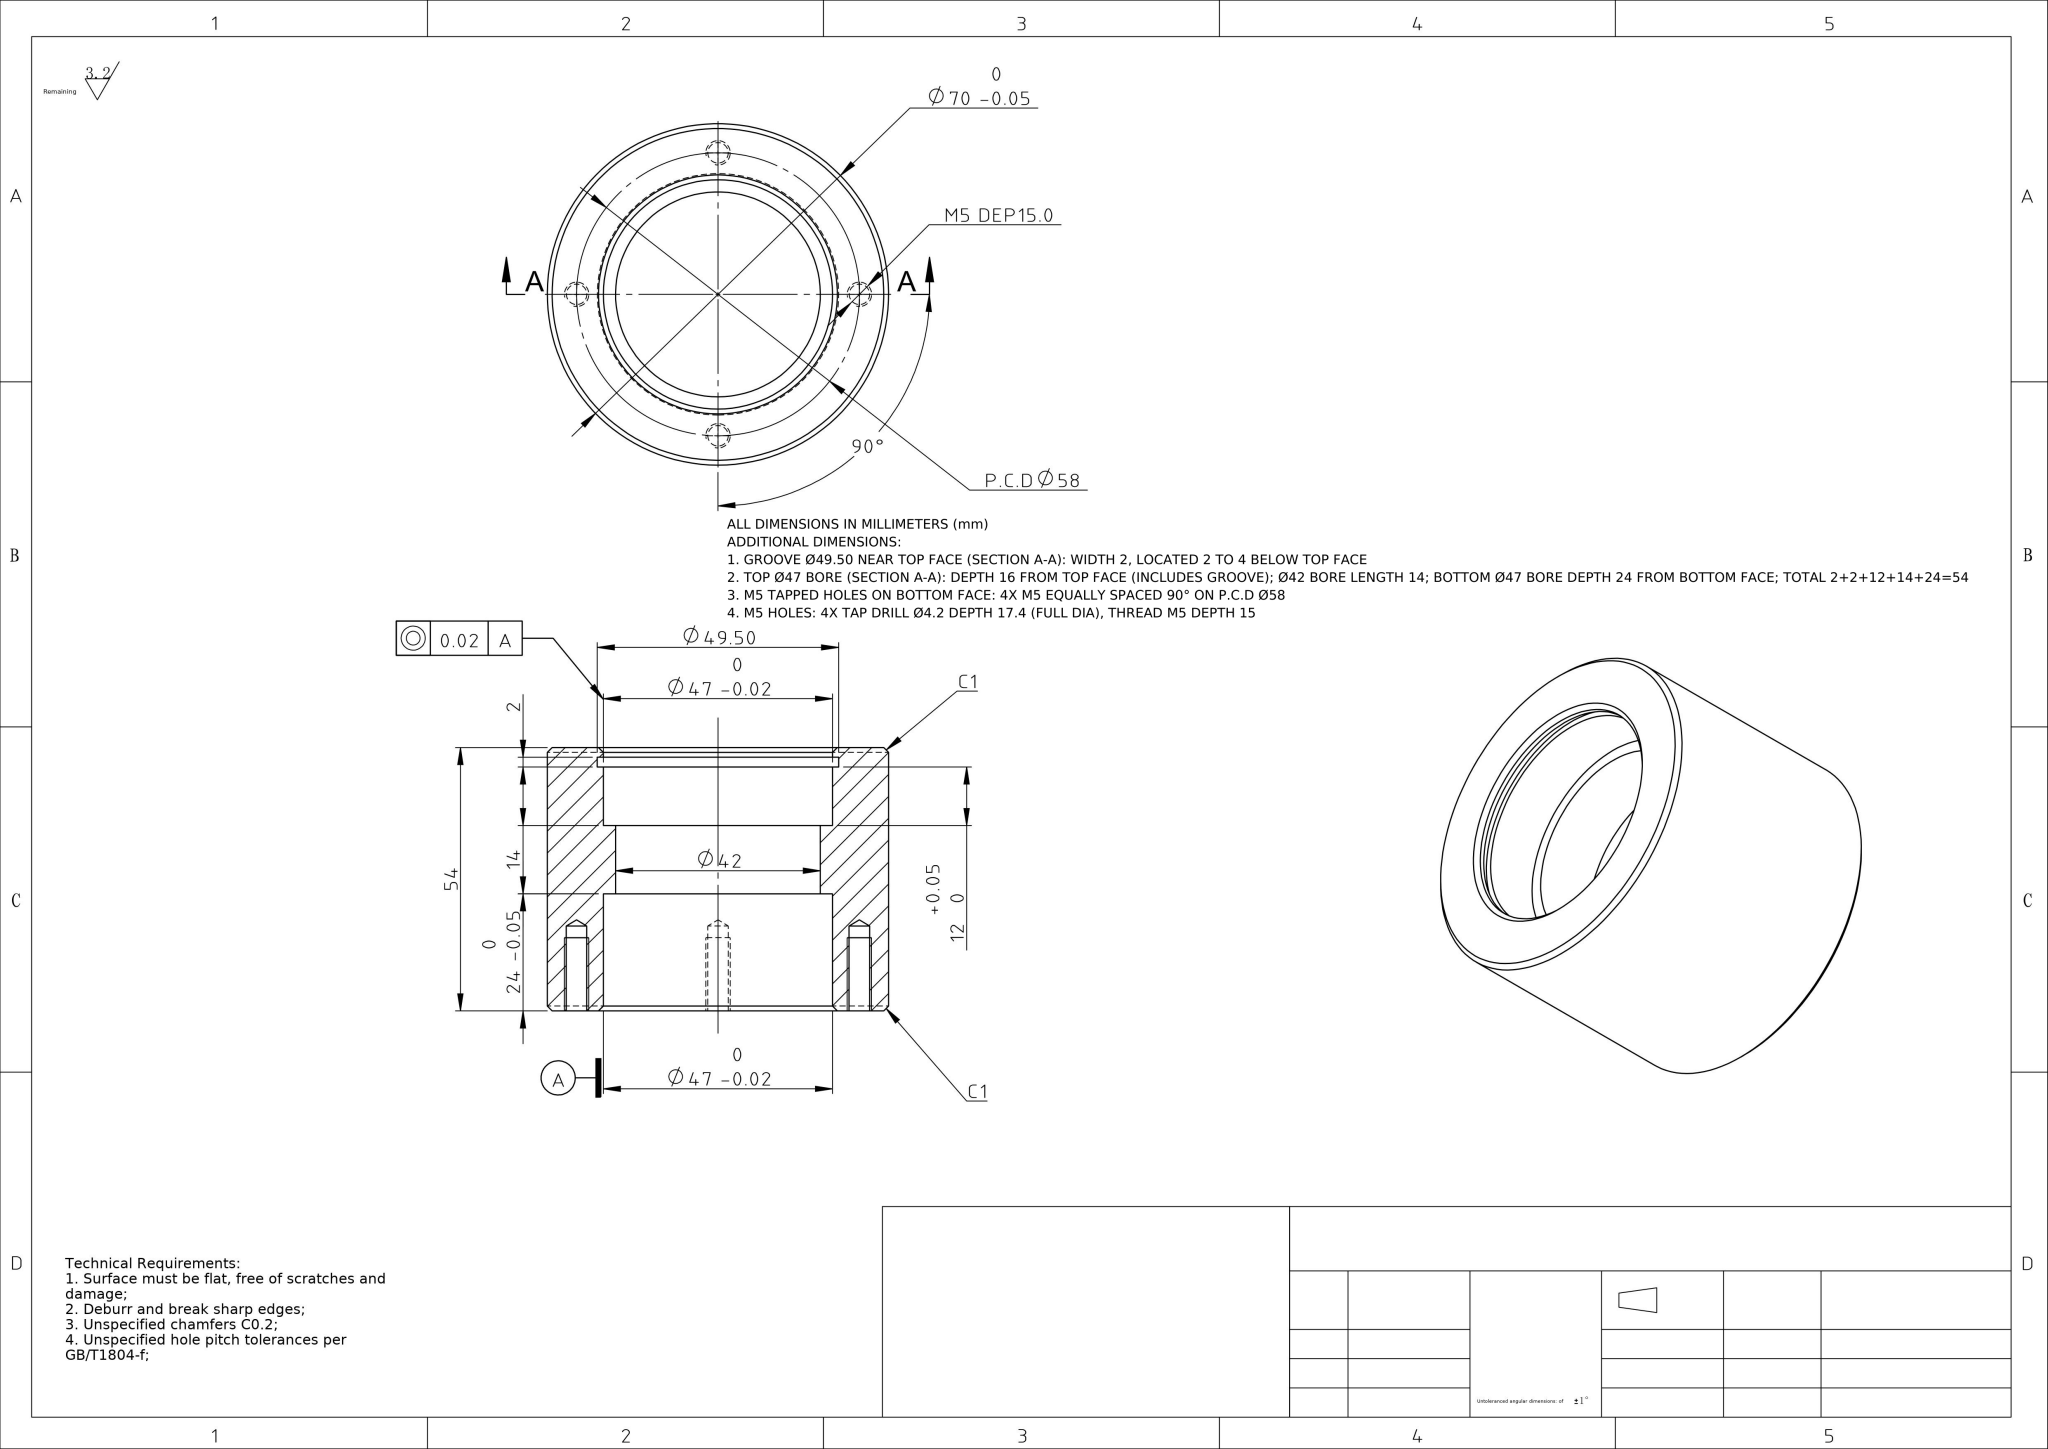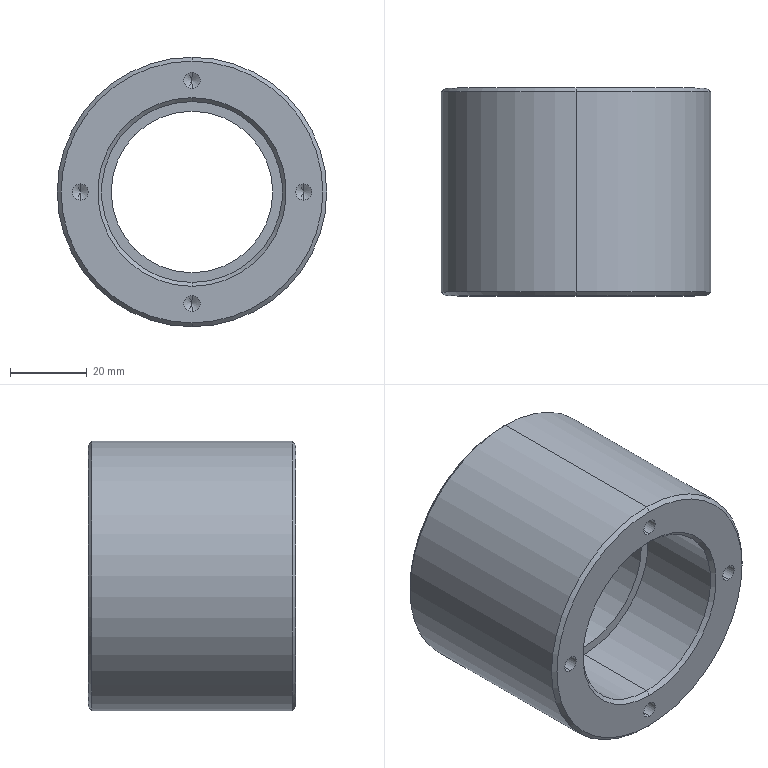Part | NX | mm | 1 solid | 42 faces | box 70 x 54 x 70 mm | volume 117288 mm3 | cylinder 20 | cone 16 | plane 6 | commonest cylinder face diameters 4.2 x8 47 x6 49.5 x2 42 x2 70 x2